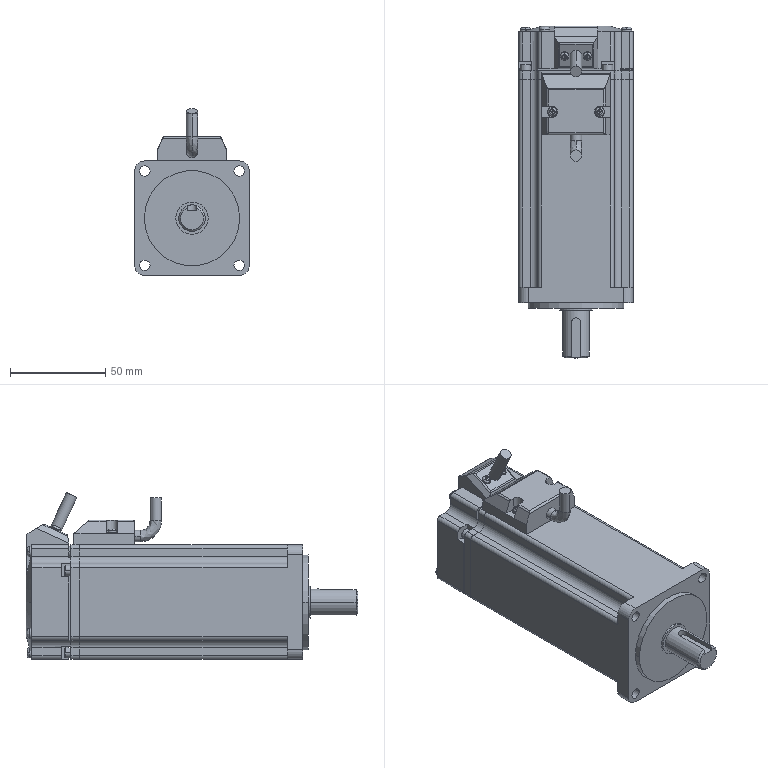Component | SolidWorks | HZ022-X-Axis-MS-60ST-M01330-20P4(Servo400W)-1 | 1 solid | 446 faces | volume 489726 mm3 | plane 283 | cylinder 123 | cone 22 | spline 18 | commonest cylinder face diameters 4 x25 5.5 x24 6 x24 8 x12 2 x11 4.5 x8 5 x5 20 x4 | material 45